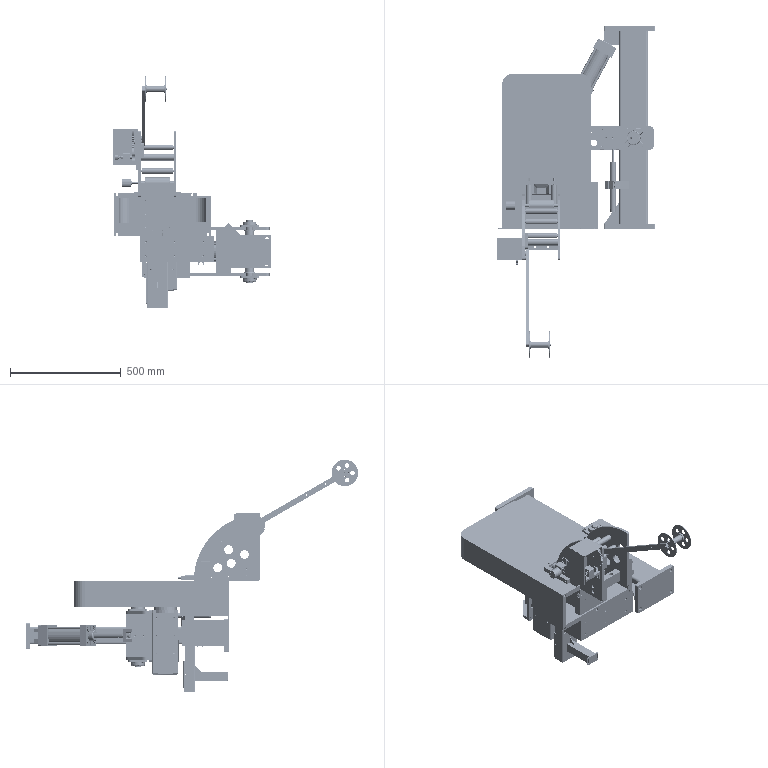Assembly | SolidWorks | mm | 77 component files | 136 solids | 6443 faces | box 714.5 x 1500.09 x 1051.5 mm | volume 27815565 mm3 | plane 2410 | cylinder 2260 | spline 1001 | cone 424 | torus 236 | sphere 112 | commonest cylinder face diameters 5 x141 9 x120 6.8 x118 20 x108 107 x105 102.497 x105 6 x102 4.2 x90
Bill of materials:
320SawBlade | 1 |  | Thin flat circular disc with evenly spaced small teeth or notches around the outer edge and a round hole in the center.
A | 1 |  | Sheet-metal hollow rectangular housing in an L shape (plan view). One end is open with a perimeter flange carrying slotted mounting holes. A long arm runs off to one side and ends in a rounded corner.
B | 1 |  | Sheet-metal shell that wraps a rectangular volume: top panel, two side walls and a partial bottom panel. One end is open, and the bottom has a large curved cutout. A narrow outward lip runs along one lower edge.
CoverPlate | 1 |  | Sheet-metal U-channel: a large flat web with two narrow side flanges bent at roughly 90 degrees. Each flange has one elongated slot.
GuideSlot | 1 |  | Welded or bent sheet bracket. An upright U-channel has a rectangular window near the top. A horizontal arm sticks out from its web, with a triangular gusset underneath and a small end plate carrying two slots.
TransitionPlate | 1 |  | Angle bracket with two legs at about 90 degrees and a rounded bend. The base leg has four round holes in a rectangular pattern, and the upright leg has a chamfered top edge.
AdjustableHydraulicBufferHR60 | 1 |  | Stepped cylindrical pin: a short larger-diameter head at one end, a long main shank, and a much smaller-diameter tip at the other end.
BladeGuard | 1 |  | Plain solid rectangular block (cuboid) with no visible holes or features.
BladeHolder | 1 |  | Flat rectangular bar with two round through-holes near its ends and small corner chamfers on one long edge.
BoltNeedleBearing | 1 |  | Turned stepped part: a large short cylindrical base with a smaller coaxial cylindrical stem. The stem has a narrow circumferential groove partway along it, and the edges are chamfered.
CB-80CylinderFixingBase(DoubleEyelet) | 1 |  | Bracket with a square flange plate, four holes near the corners and a rounded-rectangular central opening. Two parallel lugs stick out from the plate in a clevis-like form, each with an aligned round hole.
ConnectingPin1 | 1 |  | Solid cylindrical pin with chamfered ends and a narrow circumferential groove near each end.
ConnectingPin2 | 1 |  | Solid plain cylinder (pin-like) with a shallow circumferential groove near each end and small edge breaks at both end faces.
CuttingBladeCylinderGasket | 1 |  | L-section angle bracket: a rectangular horizontal plate joined along one long edge to a vertical wall, with a small raised U/C-shaped wall around a rectangular through opening near one corner of the plate.
CuttingBladeModification | 1 |  | Thin flat square plate with two parallel open-ended U-slots entering from one edge and a tapered (wedge-beveled) region along the opposite edge.
CuttingDieMount | 1 |  | Multi-wall block/frame: two parallel side walls bridged by a crossbar on top of a wider base, giving an H-like profile, with a central open cavity, many holes, and a horizontal slot cut partway into one wall.
CuttingDieMountingSeatLocatingBlock | 1 |  | Solid L-shaped block (L outline in plan) with two parallel through holes across one leg.
LocatingStrip | 1 |  | Flat bar of rectangular section with one fully rounded end and a square opposite end, with four through holes in a line along its length.
Mold01-1 | 1 |  | Rectangular block with a tapered (funnel-like) rounded-rectangle through cavity: larger opening on top, smaller opening at bottom, plus a narrow groove across one side face.
'-Mold01-2 | 1 |  | Rectangular block with a straight-walled rounded-rectangle through opening and a narrow groove across one side face; similar to a block with a tapered cavity but with straight walls.
CuttingMotorFixedAxis | 1 |  | Stepped cylindrical shaft: a larger central cylinder with a smaller-diameter coaxial journal extending from each end.
CuttingMotorFixedShaftSleeve | 2 |  | Flanged bushing: a thin wide circular flange on top of a shorter-diameter cylindrical body, with a central through bore.
CylinderMount | 1 |  | Long beam of rectangular section with rectangular end plates at both ends; each end plate has rounded corners and four corner holes; the beam has a central through hole on top, two tiny holes, and a small side tab with a hole near one end.
DamperMountingBlock | 1 |  | Bracket with an inclined arm containing a large bore and a split slot (clamp-style), a horizontal foot with two holes, and a vertical leg with a hole, joined at a filleted corner.
GraphiteCopperSleeve1 | 2 |  | Short plain cylindrical ring or spacer with a concentric through bore; axial length is less than outside diameter.
GraphiteCopperSleeve2- | 1 |  | Plain cylindrical sleeve or spacer with a concentric through bore; axial length is about equal to or slightly more than outside diameter.
ConnectingRod | 1 |  | Solid cylindrical rod or pin with small chamfers at both ends and a small central axial hole in at least one end face.
E6B2-CWZ1XEncoder | 1 |  | Cylindrical housing-like body. One end face has a concentric stepped pilot boss and a small-diameter output shaft; the shaft appears to have a flat or step near its tip. Three small holes are spaced around the end face.
EncoderRoller | 1 |  | Thin-walled cylindrical tube open at both ends with a uniform outer diameter.
EncoderSupport | 1 |  | Bent sheet-like bracket with a Z or joggle profile: two parallel flanges offset by a connecting web. One flange has two parallel obround slots; the other has a large round hole and three small holes around it. The flange ends are rounded.
GuideSeatFixingPlate | 1 |  | Rectangular block with two larger holes through the long face and two smaller holes in one end face.
GuideWheelMountingPlate | 1 |  | Flat plate shaped roughly as a quarter circle with square corners on two sides and one large arc edge. It has many through holes: several large round holes, small round holes, two small obround slots, a narrow slot from the bottom edge, and a rectangular notch at one corner. The rendering shows two identical copies side by side.
LimitPlate1 | 2 |  | Thick rectangular bar with one fully rounded (semicircular) end and one square end, with two in-line obround through slots along its length.
LimitRollerSeat | 2 |  | L-shaped bar of constant thickness with an internal corner fillet. The long leg has a small rectangular side tab or step and a small round through hole near its end; the short leg has an elongated obround through slot.
RollerAxis01 | 1 |  | Long stepped cylindrical shaft with a main central diameter and reduced-diameter shoulders and journals at both ends. One end has two steps down to a small tip; the other end has a single step.
RollerEndCap01 | 1 |  | Flanged hub or bushing: a cylindrical boss with an end chamfer joined to a larger, thin flange, with a central through bore that has a single rectangular keyway.
RollerEndCap02 | 1 |  | Flanged cylindrical bushing: thin circular flange at one end, a shorter-diameter cylindrical body with a small chamfer at the free end, and a central through bore.
'-StainlessSteelRoller(Vertical) | 2 |  | Solid stepped cylindrical shaft/pin: a long large-diameter cylinder, a short intermediate-diameter step, and a smaller-diameter pin extending from one end.
StainlessSteelRoller | 3 |  | Cylindrical roller or pin with rounded/filleted end edges and a short small-diameter stub journal at each end; the stub end face has a small conical center recess.
AdjustmentSeat.1 | 1 |  | L-shaped angle bracket of rectangular cross-section with two parallel elongated slots in the long leg and two parallel slots in the short leg.
AngleDisplacementSensor.1 | 1 |  | Stepped turned shaft/knob: large-diameter cylindrical head with a narrow circumferential groove near one end, followed by a short collar step, an intermediate-diameter section and a smaller-diameter pin with a slot across its end face.
AngleDisplacementSensorMountingPlate.1 | 1 |  | Flat plate with a rectangular lower portion and two chamfered upper corners (pentagon-like outline), one large round hole near the top and two smaller round holes near the bottom corners.
AngleDisplacementSensorNut.1 | 1 |  | Hexagonal ring of uniform thickness with a large plain circular central bore, resembling a thin hex nut shape.
AngleSensorConnectionAxis.1 | 1 |  | Stepped shaft: one end with a radial cross hole and a narrow circumferential groove nearby, a long main section, a larger-diameter collar, and an opposite end section with a flat on its side and a small axial center hole.
BearingHousing.1 | 1 |  | Rectangular block with a large central stepped (counterbored) through hole and four small through holes near the corners.
BearingHousing2.1 | 1 |  | Near-cubic block with two chamfered edges along one side and a central stepped (counterbored) through hole.
CylindricalGear105x1.1 | 1 | 45 | Thin spur gear with many fine teeth around the rim and a central bore with a single keyway notch.
CylindricalGear35x1.1 | 1 | 45 | Wide-face spur gear with roughly thirty-odd straight teeth, a large central bore, and a radial hole passing through the toothed rim.
GuideWheel | 1 |  | Spool-like body: two thin, flat, parallel circular flanges joined by a central cylindrical tube, with a short larger-diameter boss where the tube meets each flange.
GuideWheelAxis | 1 |  | Long, straight, solid cylindrical rod with a narrow ring-shaped groove near each end and a flat machined on one end.
Rolling bearings 6001 GB 276-94 | 4 |  | Ball-bearing-like annular body: concentric outer and inner rings sharing a flat-faced, equal-width profile, with a single row of about 14 spherical balls evenly spaced in the annular gap between them; open faces with no visible shield, seal or cage.
RoundNut.1 | 1 |  | Thick flat ring (annulus) with four rectangular notches evenly spaced around its outer edge.
SwingArm.1 | 1 |  | Long, thin, flat rectangular bar with small through-holes spaced along its length.
SwingRodRotationAxis.1 | 1 |  | Stepped cylindrical shaft with several coaxial diameters and a central bore at the small end.
SwingArmGuard | 1 |  | Thin-walled, sheet-like formed bracket or enclosure: flat top and bottom panels joined by vertical walls, with a perpendicular end flange that has two holes and rounded outer corners.
1 | 1 |  | Rectangular block with an extrusion-like profile: several lengthwise slots and grooves on its outer faces, two large lengthwise through-bores and four smaller corner bores.
2 | 1 |  | Rectangular plate with three parallel cylindrical rods standing out from one face: two long outer rods and a shorter central rod ending in a larger-diameter disc.
3 | 1 |  | Small block body with a lengthwise rounded rib or rod on top between two parallel rails, a stepped lower block, and a cylindrical pin pointing down from one end.
4 | 1 |  | Small block body with a lengthwise cylindrical rod on top between two parallel rails, a lower block section, and a cylindrical pin pointing down from one end.
MotorMount | 1 | Plain Carbon Steel | Plate-built U-shaped frame bracket: a square end plate with two parallel side arms extending from it, an inner cross plate with an angled gusset, and open-ended slots near the free ends of the arms.
SawingMotor | 1 |  | Rectangular housing body with a stepped cylindrical boss on one end, a rectangular box sticking out from one side, and a square flange face with four corner holes.
SC-80X130PistonRod | 1 |  | Long, slender solid cylindrical rod. One end steps down to a short, smaller-diameter cylindrical spigot, with a narrow hexagonal collar (wrench flats) next to it. The far end is plain and appears flat or slightly rounded.
SC-80X130-S-BCylinder | 1 |  | Tie-rod-style cylinder body. A cylindrical barrel sits between two rectangular end blocks, which are held by four slender rods running along the outside. One end block has a protruding round boss with a central through-bore. Its outer face has four small holes at the corners, a shallow recessed outline, and faint diagonal and centre lines.
SC-80X130-S-BCylinderY-Joint | 1 |  | U-shaped clevis block. Two parallel flat prongs with rounded ends are joined by a solid rectangular base. The prongs share one aligned cross-hole. A second hole passes through the base at right angles, opening into the slot between the prongs.
ToolHolder | 1 |  | Flat rectangular plate with small chamfered corners and four through-holes near the corners. A narrow rectangular tab or rib projects from the back face along part of its length, so the side view is T-shaped.
UCF204D1 | 2 |  | Four-bolt square flange housing with a round central boss. The boss holds an insert with an extended inner collar and a central bore. The square flange has rounded corners, four large through-holes at the corners, and diagonal ribs from the boss to the corners. A small nipple projects from the side of the boss.
Mates:
1. coincident | SC-80X130-S-BCylinder-1 face at (-106.845, 345.63, 947) dir (0.479, 0.8778, 0) | CB-80CylinderFixingBase(DoubleEyelet)-1 face at (-148.101, 368.145, 900) dir (-0.479, -0.8778, 0)
2. concentric | SC-80X130-S-BCylinder-1 face at (-184.333, 374.816, 935) dir (0.479, 0.8778, 0) r 5.5 | CB-80CylinderFixingBase(DoubleEyelet)-1 face at (-172.118, 397.2, 935) dir (0.479, 0.8778, 0) r 8.5
3. concentric | SC-80X130-S-BCylinder-1 face at (-184.333, 374.816, 865) dir (0.479, 0.8778, 0) r 5.5 | CB-80CylinderFixingBase(DoubleEyelet)-1 face at (-172.118, 397.2, 865) dir (0.479, 0.8778, 0) r 8.5
4. concentric | CylinderMount-1 face at (-132.772, 396.234, 916) dir (0, 0, -1) r 14 | CB-80CylinderFixingBase(DoubleEyelet)-1 face at (-132.772, 396.234, 865.5) dir (0, 0, 1) r 10
5. concentric | SC-80X130-S-BCylinder-1 face at (-173.49, 321.621, 900) dir (-0.479, -0.8778, 0) r 12.5 | SC-80X130PistonRod-1 face at (-355.042, -11.064, 900) dir (0.479, 0.8778, 0) r 12.5
6. distance | SC-80X130PistonRod-1 face at (-323.95, 33.486, 889.008) dir (-0.479, -0.8778, 0) | SC-80X130-S-BCylinder-1 face at (-269.296, 146.062, 900) dir (-0.479, -0.8778, 0)
7. width | MotorMount-1 face at (67.336, 5.548, 802) dir (0, 0, 1) | MotorMount-1 face at (67.336, 5.548, 998) dir (0, 0, -1) | CylinderMount-1 face at (-77.772, 438.234, 860) dir (0, 0, -1) | CylinderMount-1 face at (-77.772, 438.234, 940) dir (0, 0, 1)
8. width | 320SawBlade-1 face at (-393.08, -172.058, 1071) dir (0, 0, 1) | 320SawBlade-1 face at (-393.08, -172.058, 1068) dir (0, 0, -1) | SawingMotor-1 face at (-418.028, -170.45, 1071) dir (0, 0, -1) | SawingMotor-1 face at (-365.029, -170.559, 1068) dir (0, 0, 1)
9. concentric | SawingMotor-1 face at (-418.028, -170.45, 1100) dir (0, 0, 1) r 42.5 | 320SawBlade-1 face at (-418.028, -170.45, 909.976) dir (0, 0, -1) r 25
10. concentric | SC-80X130PistonRod-1 face at (-339.234, 17.903, 900) dir (-0.479, -0.8778, 0) r 10 | SC-80X130-S-BCylinderY-Joint-1 face at (-344.024, 9.125, 900) dir (0.479, 0.8778, 0) r 10.05
11. coincident | SC-80X130PistonRod-1 face at (-344.024, 9.125, 900) dir (-0.479, -0.8778, 0) | SC-80X130-S-BCylinderY-Joint-1 face at (-324.274, -1.653, 930) dir (0.479, 0.8778, 0)
12. width | SC-80X130-S-BCylinderY-Joint-1 face at (-364.991, -76.266, 930) dir (0, 0, 1) | SC-80X130-S-BCylinderY-Joint-1 face at (-324.274, -1.653, 870) dir (0, 0, -1) | MotorMount-1 face at (-220.272, -46.358, 885) dir (0, 0, -1) | MotorMount-1 face at (-220.272, -46.358, 915) dir (0, 0, 1)
13. concentric | MotorMount-1 face at (-372.766, -43.543, 750) dir (0, 0, 1) r 14 | SC-80X130-S-BCylinderY-Joint-1 face at (-372.766, -43.543, 930) dir (0, 0, -1) r 14
14. coincident | MotorMount-1 face at (67.336, 5.548, 1010) dir (0, 0, 1) | UCF204D1-1 face at (-54.706, -14.7, 1010) dir (0, 0, -1)
15. concentric | MotorMount-1 face at (-22.772, -46.766, 750) dir (0, 0, 1) r 15 | UCF204D1-1 face at (-22.772, -46.766, 1010) dir (0, 0, -1) r 10
16. concentric | CylinderMount-1 face at (-22.772, -46.766, 824) dir (0, 0, 1) r 19 | MotorMount-1 face at (-22.772, -46.766, 750) dir (0, 0, 1) r 15
17. concentric | MotorMount-1 face at (-54.706, -14.7, 1010) dir (0, 0, 1) r 4.25 | UCF204D1-1 face at (-54.706, -14.7, 1019.35) dir (0, 0, -1) r 6
18. coincident | MotorMount-1 face at (67.336, 5.548, 790) dir (0, 0, -1) | UCF204D1-2 face at (9.294, -14.832, 790) dir (0, 0, 1)
19. concentric | MotorMount-1 face at (9.294, -14.832, 1010) dir (0, 0, 1) r 4.25 | UCF204D1-2 face at (9.294, -14.832, 780.65) dir (0, 0, 1) r 6
20. concentric | MotorMount-1 face at (-54.706, -14.7, 1010) dir (0, 0, 1) r 4.25 | UCF204D1-2 face at (-54.706, -14.7, 780.65) dir (0, 0, 1) r 6
21. concentric | CylinderMount-1 face at (-22.772, -46.766, 824) dir (0, 0, 1) r 19 | CuttingMotorFixedAxis-1 face at (-22.772, -46.766, 442.271) dir (0, 0, -1) r 19
22. width | CuttingMotorFixedAxis-1 face at (-22.772, -36.766, 806) dir (0, 0, -1) | CuttingMotorFixedAxis-1 face at (-22.772, -27.766, 994) dir (0, 0, 1) | CylinderMount-1 face at (-77.772, 438.234, 940) dir (0, 0, 1) | CylinderMount-1 face at (-77.772, 438.234, 860) dir (0, 0, -1)
23. coincident | CuttingMotorFixedAxis-1 face at (-22.772, -36.766, 806) dir (0, 0, -1) | CuttingMotorFixedShaftSleeve-1 face at (-12.772, -46.766, 806) dir (0, 0, 1)
24. concentric | CuttingMotorFixedAxis-1 face at (-22.772, -46.766, 442.271) dir (0, 0, -1) r 10 | CuttingMotorFixedShaftSleeve-1 face at (-22.772, -46.766, -457.669) dir (0, 0, -1) r 15
25. coincident | CuttingMotorFixedAxis-1 face at (-22.772, -27.766, 994) dir (0, 0, 1) | CuttingMotorFixedShaftSleeve-2 face at (-32.009, -50.596, 994) dir (0, 0, -1)
26. concentric | CuttingMotorFixedAxis-1 face at (-22.772, -46.766, 442.271) dir (0, 0, -1) r 10 | CuttingMotorFixedShaftSleeve-2 face at (-22.772, -46.766, 2257.669) dir (0, 0, 1) r 15
27. width | ConnectingPin1-1 face at (-372.766, -43.543, 933) dir (0, 0, 1) | ConnectingPin1-1 face at (-372.766, -43.543, 867) dir (0, 0, -1) | SC-80X130-S-BCylinderY-Joint-1 face at (-324.274, -1.653, 870) dir (0, 0, -1) | SC-80X130-S-BCylinderY-Joint-1 face at (-364.991, -76.266, 930) dir (0, 0, 1)
28. concentric | SC-80X130-S-BCylinderY-Joint-1 face at (-372.766, -43.543, 930) dir (0, 0, -1) r 14 | ConnectingPin1-1 face at (-372.766, -43.543, 933) dir (0, 0, -1) r 10
29. concentric | SC-80X130-S-BCylinderY-Joint-1 face at (-372.766, -43.543, 930) dir (0, 0, -1) r 14 | GraphiteCopperSleeve1-1 face at (-372.766, -43.543, 930) dir (0, 0, -1) r 14
30. coincident | SC-80X130-S-BCylinderY-Joint-1 face at (-331.459, -14.82, 915) dir (0, 0, -1) | GraphiteCopperSleeve1-1 face at (-372.766, -43.543, 915) dir (0, 0, -1)
31. concentric | SC-80X130-S-BCylinderY-Joint-1 face at (-372.766, -43.543, 930) dir (0, 0, -1) r 14 | GraphiteCopperSleeve1-2 face at (-372.766, -43.543, 885) dir (0, 0, -1) r 14
32. coincident | SC-80X130-S-BCylinderY-Joint-1 face at (-364.991, -76.266, 885) dir (0, 0, 1) | GraphiteCopperSleeve1-2 face at (-372.766, -43.543, 885) dir (0, 0, 1)
33. coincident | MotorMount-1 face at (-220.272, -46.358, 885) dir (0, 0, -1) | GraphiteCopperSleeve2--1 face at (-372.766, -43.543, 885) dir (0, 0, -1)
34. concentric | MotorMount-1 face at (-372.766, -43.543, 750) dir (0, 0, 1) r 14 | GraphiteCopperSleeve2--1 face at (-372.766, -43.543, 915) dir (0, 0, -1) r 14
35. coincident | MotorMount-1 face at (67.336, 5.548, 998) dir (0, 0, -1) | BoltNeedleBearing-1 face at (-115.847, -83.074, 998) dir (0, 0, 1)
36. concentric | MotorMount-1 sketch segment at (-115.847, -83.074, 1010) dir (0, 0, 1) r 5.5 | BoltNeedleBearing-1 face at (-115.847, -83.074, 1021) dir (0, 0, -1) r 5
37. distance | CylinderMount-1 face at (-41.272, -436.766, 900) dir (0, 1, 0) | AdjustableHydraulicBufferHR60-1 face at (-115.446, -379.666, 991.405) dir (0, -1, 0)
38. concentric | CylinderMount-1 face at (-25.272, -249.266, 940) dir (0, 0, 1) r 2.5 | DamperMountingBlock-2 face at (-25.272, -249.266, 955) dir (0, 0, 1) r 3.5
39. coincident | CylinderMount-1 face at (-77.772, 438.234, 940) dir (0, 0, 1) | DamperMountingBlock-2 face at (-7.272, -241.766, 940) dir (0, 0, -1)
40. concentric | CylinderMount-1 face at (-25.272, -269.266, 940) dir (0, 0, 1) r 2.5 | DamperMountingBlock-2 face at (-25.272, -269.266, 955) dir (0, 0, 1) r 5.5
41. concentric | AdjustableHydraulicBufferHR60-1 face at (-115.446, -156.166, 991.405) dir (0, -1, 0) r 12 | DamperMountingBlock-2 face at (-115.446, -241.766, 991.405) dir (0, -1, 0) r 12
42. concentric | CB-80CylinderFixingBase(DoubleEyelet)-1 face at (-132.772, 396.234, 865.5) dir (0, 0, 1) r 10 | ConnectingPin2-1 face at (-132.772, 396.234, 937.5) dir (0, 0, -1) r 10
43. width | ConnectingPin2-1 face at (-132.772, 396.234, 937.5) dir (0, 0, 1) | ConnectingPin2-1 face at (-132.772, 396.234, 862.5) dir (0, 0, -1) | CB-80CylinderFixingBase(DoubleEyelet)-1 face at (-143.049, 425.766, 868) dir (0, 0, -1) | CB-80CylinderFixingBase(DoubleEyelet)-1 face at (-143.049, 425.766, 932) dir (0, 0, 1)
44. coincident | MotorMount-1 face at (-220.405, -110.858, 900) dir (-0.002066, -1, 0) | SawingMotor-1 face at (-352.905, -110.584, 723) dir (0.002066, 1, 0)
45. distance | SawingMotor-1 face at (-485.911, -113.309, 723) dir (-1, 0.002066, 0) | MotorMount-1 face at (-507.904, -110.264, 780) dir (-1, 0.002066, 0)
46. distance | SawingMotor-1 face at (-377.915, -115.532, 1015) dir (0, 0, 1) | MotorMount-1 face at (-327.905, -110.636, 1017) dir (0, 0, 1)
47. coincident | AA-1/A-1 face at (-636.772, -452.766, 968.5) dir (0, 0, -1) | CuttingBladeCylinderGasket-1 face at (-361.772, -326.766, 968.5) dir (0, 0, 1)
48. width | CuttingBladeModification-1 face at (-464.272, -249.266, 895.2) dir (0, 1, 0) | CuttingBladeModification-1 face at (-464.272, -314.266, 895.2) dir (0, -1, 0) | CuttingDie-1/-Mold01-2-1 face at (-461.272, -261.766, 1002) dir (0, -1, 0) | CuttingDie-1/-Mold01-2-1 face at (-461.272, -301.766, 1002) dir (0, 1, 0)
49. width | BladeGuard-1 face at (-464.272, -246.766, 910.2) dir (0, 1, 0) | BladeGuard-1 face at (-464.272, -316.766, 910.2) dir (0, -1, 0) | CuttingDie-1/-Mold01-2-1 face at (-461.272, -261.766, 1002) dir (0, -1, 0) | CuttingDie-1/-Mold01-2-1 face at (-461.272, -301.766, 1002) dir (0, 1, 0)
50. parallel | CuttingDie-1/-Mold01-2-1 face at (-464.272, -298.766, 1002) dir (1, 0, 0) | BladeGuard-1 face at (-464.272, -316.766, 910.2) dir (1, 0, 0)
51. coincident | CuttingDie-1/-Mold01-2-1 face at (-464.272, -298.766, 1002) dir (1, 0, 0) | BladeGuard-1 face at (-464.272, -316.766, 910.2) dir (1, 0, 0)
52. coincident | CuttingBladeCylinderGasket-1 face at (-479.272, -246.766, 968.5) dir (1, 0, 0) | BladeGuard-1 face at (-479.272, -316.766, 910.2) dir (-1, 0, 0)
53. width | BladeGuard-1 face at (-471.772, -281.766, 910.2) dir (0, 0, 1) | BladeGuard-1 face at (-471.772, -281.766, 880.2) dir (0, 0, -1) | CuttingBladeModification-1 face at (-404.772, -249.266, 894.2) dir (0, 0, -1) | CuttingBladeModification-1 face at (-404.772, -249.266, 896.2) dir (0, 0, 1)
54. parallel | ToolHolder-1 face at (-404.772, -327.766, 894.5) dir (-1, 0, 0) | CuttingBladeModification-1 face at (-404.772, -249.266, 894.2) dir (1, 0, 0)
55. coincident | ToolHolder-1 face at (-404.772, -327.766, 894.5) dir (-1, 0, 0) | CuttingBladeModification-1 face at (-404.772, -249.266, 894.2) dir (1, 0, 0)
56. coincident | ToolHolder-1 face at (-392.772, -327.766, 894.5) dir (1, 0, 0) | MGPM63-55-M9NV_0_1_0-1/2-1 face at (-392.772, -327.766, 894.5) dir (-1, 0, 0)
57. concentric | MGPM63-55-M9NV_0_1_0-1/2-1 face at (-384.772, -392.766, 869.5) dir (1, 0, 0) r 4.188 | ToolHolder-1 face at (-404.772, -392.766, 869.5) dir (-1, 0, 0) r 5.5
58. coincident | AA-1/A-1 face at (-484.272, -253.766, 1166.5) dir (0, -1, 0) | GuideMechanism-1/LimitRollerSeat-2 face at (-413.272, -253.766, 1171.5) dir (0, -1, 0)
59. coincident | AA-1/A-1 face at (-616.772, 243.234, 1146.5) dir (0, 0, 1) | GuideMechanism-1/GuideWheelMountingPlate-1 face at (-353.272, -298.766, 1146.5) dir (0, 0, -1)
60. coincident | A-1 face at (322.308, 345.256, 549.124) dir (0, 0, 1) | TransitionPlate-1 face at (100.308, -237.257, 549.124) dir (0, 0, -1)
61. coincident | A-1 face at (189.808, -201.744, 525.124) dir (0, 1, 0) | TransitionPlate-1 face at (100.308, -201.744, 549.124) dir (0, -1, 0)
62. width | TransitionPlate-1 face at (189.308, -202.744, 548.124) dir (1, 0, 0) | TransitionPlate-1 face at (100.308, -202.744, 552.124) dir (-1, 0, 0) | A-1 face at (189.808, -151.744, 525.124) dir (-1, 0, 0) | A-1 face at (99.808, -151.744, 525.124) dir (1, 0, 0)
63. width | GuideSlot-1 face at (192.808, -151.744, 838.124) dir (1, 0, 0) | GuideSlot-1 face at (96.808, -151.744, 838.124) dir (-1, 0, 0) | A-1 face at (99.808, -151.744, 525.124) dir (1, 0, 0) | A-1 face at (189.808, -151.744, 525.124) dir (-1, 0, 0)
64. coincident | GuideSlot-1 face at (189.808, -151.744, 838.124) dir (0, 1, 0) | CoverPlate-1 face at (144.808, -151.744, 968.124) dir (0, -1, 0)
65. width | CoverPlate-1 face at (96.808, -150.244, 968.124) dir (1, 0, 0) | CoverPlate-1 face at (192.808, -150.244, 968.124) dir (-1, 0, 0) | GuideSlot-1 face at (96.808, -151.744, 838.124) dir (-1, 0, 0) | GuideSlot-1 face at (192.808, -151.744, 838.124) dir (1, 0, 0)
66. distance | A-1 face at (322.308, 345.256, 703.124) dir (0, 0, 1) | CoverPlate-1 face at (97.808, -151.744, 908.124) dir (0, 0, -1)
67. coincident | A-1 face at (122.308, 345.256, 624.124) dir (0, 1, 0) | B-1 face at (322.308, 345.256, 663.124) dir (0, 1, 0)
68. coincident | A-1 face at (92.308, -107.744, 699.124) dir (1, 0, 0) | B-1 face at (92.308, 103.756, 604.124) dir (-1, 0, 0)
69. coincident | A-1 face at (322.308, 345.256, 545.124) dir (0, 0, -1) | B-1 face at (322.308, -137.744, 545.124) dir (0, 0, -1)
70. parallel | A-1 face at (322.308, 345.256, 545.124) dir (0, 0, -1) | AA plane at (0, 0, 0) dir (0, 0, 1)
71. parallel | A-1 face at (122.308, -354.744, 624.124) dir (0, -1, 0) | AA plane at (0, 0, 0) dir (0, 1, 0)
72. distance | GuideSlot-1 face at (100.808, -200.744, 838.124) dir (0, 0, -1) | A-1 face at (322.308, 345.256, 703.124) dir (0, 0, 1)
73. coincident | CuttingDieMount-1 face at (49.289, -80.571, 190) dir (1, 0, 0) | CuttingDieMountingSeatLocatingBlock-1 face at (49.289, -50.571, 120.5) dir (1, 0, 0)
74. coincident | CuttingDieMount-1 face at (49.289, -95.571, 102.5) dir (0, 0, -1) | CuttingDieMountingSeatLocatingBlock-1 face at (49.289, -95.571, 102.5) dir (0, 0, 1)
75. coincident | CuttingDieMount-1 face at (49.289, -65.571, 102.5) dir (0, 1, 0) | CuttingDieMountingSeatLocatingBlock-1 face at (49.289, -65.571, 102.5) dir (0, -1, 0)
76. coincident | CuttingDieMount-1 face at (29.289, -95.571, 102.5) dir (-1, 0, 0) | LocatingStrip-1 face at (29.289, -95.571, 282.5) dir (1, 0, 0)
77. coincident | CuttingDieMount-1 face at (4.289, -83.571, 102.5) dir (0, -1, 0) | LocatingStrip-1 face at (29.289, -83.571, 282.5) dir (0, 1, 0)
78. coincident | CuttingDieMount-1 face at (49.289, -95.571, 102.5) dir (0, 0, -1) | LocatingStrip-1 face at (16.789, -89.571, 102.5) dir (0, 0, -1)
79. coincident | CuttingDieMount-1 face at (-20.711, 54.429, 190) dir (0, 1, 0) | -Mold01-2-1 face at (-55.711, 54.429, 190) dir (0, -1, 0)
80. width | -Mold01-2-1 face at (-53.211, 54.429, 142) dir (-1, 0, 0) | -Mold01-2-1 face at (-58.211, 54.429, 142) dir (1, 0, 0) | CuttingDieMount-1 face at (-58.211, 24.429, 139.5) dir (-1, 0, 0) | CuttingDieMount-1 face at (-53.211, 24.429, 139.5) dir (1, 0, 0)
81. coincident | CuttingDieMount-1 face at (-90.711, 99.429, 142) dir (0, 0, 1) | -Mold01-2-1 face at (-88.211, 119.429, 142) dir (0, 0, -1)
82. coincident | CuttingDieMount-1 face at (-20.711, 54.429, 190) dir (0, 1, 0) | Mold01-1-3 face at (14.289, 54.429, 190) dir (0, -1, 0)
83. width | Mold01-1-3 face at (11.789, 54.429, 142) dir (1, 0, 0) | Mold01-1-3 face at (16.789, 54.429, 142) dir (-1, 0, 0) | CuttingDieMount-1 face at (11.789, 24.429, 139.5) dir (-1, 0, 0) | CuttingDieMount-1 face at (16.789, 24.429, 139.5) dir (1, 0, 0)
84. coincident | CuttingDieMount-1 face at (-90.711, 99.429, 142) dir (0, 0, 1) | Mold01-1-3 face at (-18.211, 119.429, 142) dir (0, 0, -1)
85. width | GuideSeatFixingPlate-1 face at (16.59, -118.843, 215) dir (1, 0, 0) | GuideSeatFixingPlate-1 face at (-131.41, -118.843, 215) dir (-1, 0, 0) | GuideWheelMountingPlate-1 face at (16.59, -163.843, 150) dir (-1, 0, 0) | GuideWheelMountingPlate-1 face at (-131.41, -163.843, 150) dir (1, 0, 0)
86. distance | GuideWheelMountingPlate-1 face at (28.59, 136.157, 150) dir (0, 0, -1) | GuideSeatFixingPlate-1 face at (-57.41, -103.843, 165) dir (0, 0, -1)
87. distance | GuideWheelMountingPlate-1 face at (28.59, -163.843, 150) dir (0, -1, 0) | GuideSeatFixingPlate-1 face at (16.59, -118.843, 215) dir (0, -1, 0)
88. concentric | GuideWheelMountingPlate-1 face at (20.59, -83.843, 330) dir (1, 0, 0) r 7 | ConnectingRod-1 face at (16.59, -83.843, 330) dir (-1, 0, 0) r 15
89. coincident | GuideWheelMountingPlate-1 face at (16.59, -163.843, 150) dir (-1, 0, 0) | ConnectingRod-1 face at (16.59, -83.843, 330) dir (1, 0, 0)
90. width | LimitRollerSeat-1 face at (-123.41, 128.657, 175) dir (0, 0, 1) | LimitRollerSeat-1 face at (-123.41, 128.657, 155) dir (0, 0, -1) | GuideWheelMountingPlate-1 face at (28.59, 154.061, 155) dir (0, 0, 1) | GuideWheelMountingPlate-1 face at (28.59, 154.061, 175) dir (0, 0, -1)
91. coincident | GuideWheelMountingPlate-1 face at (-143.41, -163.843, 150) dir (-1, 0, 0) | LimitRollerSeat-1 face at (-143.41, 86.157, 155) dir (1, 0, 0)
92. coincident | GuideWheelMountingPlate-1 face at (28.59, -163.843, 150) dir (1, 0, 0) | LimitRollerSeat-2 face at (28.59, 86.157, 175) dir (-1, 0, 0)
93. coincident | GuideWheelMountingPlate-1 face at (28.59, 154.061, 155) dir (0, 0, 1) | LimitRollerSeat-2 face at (8.59, 128.657, 155) dir (0, 0, -1)
94. coincident | GuideWheelMountingPlate-1 face at (28.59, 66.157, 155) dir (0, 1, 0) | LimitRollerSeat-1 face at (-163.41, 66.157, 175) dir (0, -1, 0)
95. coincident | GuideWheelMountingPlate-1 face at (28.59, 66.157, 155) dir (0, 1, 0) | LimitRollerSeat-2 face at (48.59, 66.157, 155) dir (0, -1, 0)
96. width | -StainlessSteelRoller(Vertical)-7 face at (-130.184, 181.157, 169) dir (0, 0, 1) | -StainlessSteelRoller(Vertical)-7 face at (-125.226, 181.157, 161) dir (0, 0, -1) | LimitRollerSeat-1 face at (-93.41, 41.157, 161) dir (0, 0, 1) | LimitRollerSeat-1 face at (-93.41, 41.157, 169) dir (0, 0, -1)
97. coincident | LimitRollerSeat-1 face at (-83.41, 181.157, 155) dir (0, -1, 0) | -StainlessSteelRoller(Vertical)-7 face at (-114.91, 181.157, 165) dir (0, 1, 0)
98. coincident | LimitRollerSeat-2 face at (-21.41, 41.157, 161) dir (0, 0, 1) | -StainlessSteelRoller(Vertical)-8 face at (15.363, 181.157, 161) dir (0, 0, -1)
99. coincident | LimitRollerSeat-2 face at (-31.41, 181.157, 175) dir (0, -1, 0) | -StainlessSteelRoller(Vertical)-8 face at (0.08965, 181.157, 165) dir (0, 1, 0)
100. distance | -StainlessSteelRoller(Vertical)-7 plane at (-114.91, 125.157, 165) dir (-1, 0, 0) | -StainlessSteelRoller(Vertical)-8 plane at (0.08965, 125.157, 165) dir (1, 0, 0)
101. width | -StainlessSteelRoller(Vertical)-7 plane at (-114.91, 125.157, 165) dir (-1, 0, 0) | -StainlessSteelRoller(Vertical)-8 plane at (0.08965, 125.157, 165) dir (1, 0, 0) | LimitRollerSeat-2 face at (48.59, 191.157, 155) dir (1, 0, 0) | LimitRollerSeat-1 face at (-163.41, 191.157, 175) dir (-1, 0, 0)
102. concentric | GuideWheelMountingPlate-1 face at (-131.41, 56.894, 267.368) dir (-1, 0, 0) r 3 | StainlessSteelRoller-3 face at (-277.595, 56.894, 267.368) dir (-1, 0, 0) r 12.5
103. concentric | GuideWheelMountingPlate-1 face at (-131.41, 9.821, 329.835) dir (-1, 0, 0) r 3 | StainlessSteelRoller-4 face at (-277.595, 9.821, 329.835) dir (-1, 0, 0) r 12.5
104. concentric | GuideWheelMountingPlate-1 face at (-131.41, -54.25, 374.699) dir (-1, 0, 0) r 3 | StainlessSteelRoller-2 face at (-277.595, -54.25, 374.699) dir (-1, 0, 0) r 12.5
105. coincident | GuideWheelMountingPlate-1 face at (-131.41, -163.843, 150) dir (1, 0, 0) | StainlessSteelRoller-4 face at (-131.41, 9.821, 329.835) dir (-1, 0, 0)
106. coincident | StainlessSteelRoller-2 face at (12.59, -41.758, 374.249) dir (1, 0, 0) | StainlessSteelRoller-4 face at (12.59, 21.948, 326.801) dir (1, 0, 0)
107. coincident | GuideWheelMountingPlate-1 face at (-143.41, -163.843, 150) dir (-1, 0, 0) | SwingArm-1/AdjustmentSeat.1-1 face at (-143.41, -116.343, 269.95) dir (1, 0, 0)
108. distance | GuideWheelMountingPlate-1 face at (-131.41, 136.157, 150) dir (0, 0, -1) | SwingArm-1/AdjustmentSeat.1-1 face at (-153.41, -116.343, 269.95) dir (0, 0, -1)
109. concentric | GuideWheelMountingPlate-1 face at (-143.41, 82.359, 213.412) dir (1, 0, 0) r 7.5 | EncoderRoller-1 face at (-428.401, 82.359, 213.412) dir (-1, 0, 0) r 26
110. concentric | EncoderRoller-1 face at (-428.401, 82.359, 213.412) dir (-1, 0, 0) r 26 | RollerAxis01-1 face at (466.097, 82.359, 213.412) dir (1, 0, 0) r 7.5
111. concentric | EncoderRoller-1 edge at (-109.91, 82.359, 213.412) dir (-1, 0, 0) r 26 | RollerEndCap02-1 face at (-114.91, 82.359, 213.412) dir (-1, 0, 0) r 22.5
112. coincident | EncoderRoller-1 face at (-109.91, 77.902, 209.395) dir (-1, 0, 0) | RollerEndCap02-1 face at (-109.91, 59.859, 213.412) dir (1, 0, 0)
113. concentric | EncoderRoller-1 face at (-19.91, 82.359, 213.412) dir (1, 0, 0) r 22.5 | RollerEndCap01-1 face at (0.08965, 82.359, 213.412) dir (1, 0, 0) r 22.5
114. coincident | EncoderRoller-1 face at (-4.91, 63.047, 196.003) dir (1, 0, 0) | RollerEndCap01-1 face at (-4.91, 104.859, 213.412) dir (-1, 0, 0)
115. coincident | RollerAxis01-1 face at (-114.91, 82.359, 213.412) dir (-1, 0, 0) | RollerEndCap02-1 face at (-114.91, 56.359, 213.412) dir (-1, 0, 0)
116. width | RollerEndCap01-1 face at (0.08965, 108.359, 213.412) dir (1, 0, 0) | RollerEndCap02-1 face at (-114.91, 56.359, 213.412) dir (-1, 0, 0) | GuideWheelMountingPlate-1 face at (-143.41, -163.843, 150) dir (-1, 0, 0) | GuideWheelMountingPlate-1 face at (28.59, -163.843, 150) dir (1, 0, 0)
117. concentric | RollerAxis01-1 face at (-141.41, 82.359, 213.412) dir (-1, 0, 0) r 3 | E6B2-CWZ1XEncoder-1 face at (-158.41, 82.359, 213.412) dir (-1, 0, 0) r 3
118. parallel | GuideWheelMountingPlate-1 face at (-131.41, -163.843, 150) dir (0, -1, 0) | E6B2-CWZ1XEncoder-1 face at (-168.41, 84.359, 215.648) dir (0, 1, 0)
119. coincident | E6B2-CWZ1XEncoder-1 face at (-178.41, 82.359, 213.412) dir (1, 0, 0) | EncoderSupport-1 face at (-178.41, 102.359, 193.412) dir (-1, 0, 0)
120. concentric | E6B2-CWZ1XEncoder-1 face at (-178.41, 82.359, 213.412) dir (-1, 0, 0) r 20 | EncoderSupport-1 face at (-168.41, 82.359, 213.412) dir (-1, 0, 0) r 10.1
121. parallel | GuideWheelMountingPlate-1 face at (-131.41, -163.843, 150) dir (0, -1, 0) | EncoderSupport-1 face at (-178.41, 102.359, 237.675) dir (0, 1, 0)
122. distance | RollerAxis01-1 face at (-156.41, 89.324, 216.194) dir (-1, 0, 0) | E6B2-CWZ1XEncoder-1 face at (-158.41, 82.359, 213.412) dir (1, 0, 0)
123. distance | GuideWheelMountingPlate-1 face at (-131.41, -163.843, 150) dir (0, -1, 0) | SwingArm-1/BearingHousing.1-1 face at (-143.41, -153.843, 430) dir (0, -1, 0)
124. coincident | GuideWheelMountingPlate-1 face at (-131.41, -163.843, 150) dir (1, 0, 0) | LimitPlate1-1 face at (-131.41, -153.843, 360.5) dir (-1, 0, 0)
125. coincident | GuideWheelMountingPlate-1 face at (-131.41, -163.843, 150) dir (0, -1, 0) | LimitPlate1-1 face at (-116.41, -163.843, 395.5) dir (0, -1, 0)
126. distance | LimitPlate1-1 face at (-116.41, -163.843, 325.5) dir (0, 0, -1) | GuideWheelMountingPlate-1 face at (-131.41, 136.157, 150) dir (0, 0, -1)
127. coincident | GuideWheelMountingPlate-1 face at (-131.41, -163.843, 150) dir (1, 0, 0) | LimitPlate1-2 face at (-131.41, -78.843, 415) dir (-1, 0, 0)
128. distance | GuideWheelMountingPlate-1 face at (-131.41, -163.843, 150) dir (0, -1, 0) | LimitPlate1-2 face at (-116.41, -43.843, 405) dir (0, 1, 0)
129. distance | LimitPlate1-2 face at (-116.41, -113.843, 405) dir (0, 0, -1) | GuideWheelMountingPlate-1 face at (-131.41, 136.157, 150) dir (0, 0, -1)
130. angle | GuideWheelMountingPlate-1 face at (-131.41, -163.843, 150) dir (0, -1, 0) | SwingArm-1/SwingArm.1-1 face at (-124.91, -560.115, 631.675) dir (0, -0.5, -0.866)
131. coincident | GuideWheelMountingPlate-1 face at (-143.41, -163.843, 150) dir (-1, 0, 0) | SwingArmGuard-1 face at (-143.41, -55.343, 376.5) dir (1, 0, 0)
132. distance | SwingArmGuard-1 face at (-144.91, -55.343, 455) dir (0, 0, -1) | GuideWheelMountingPlate-1 face at (-131.41, -163.843, 150) dir (-1, 0, 0) r 300
133. coincident | GuideWheelMountingPlate-1 face at (-131.41, -163.843, 150) dir (0, -1, 0) | SwingArmGuard-1 face at (-145.647, -163.843, 456.5) dir (0, -1, 0)
134. concentric | BearingHousing2.1-1 face at (-11.692, 4.23, 47) dir (0, 0, 1) r 14 | Rolling bearings 6001 GB 276-94-1 face at (-11.692, 4.23, 44.029) dir (0, 0, -1) r 6
135. coincident | BearingHousing2.1-1 face at (-11.692, 4.23, 47) dir (0, 0, 1) | Rolling bearings 6001 GB 276-94-1 face at (-11.692, 18.23, 47) dir (0, 0, -1)
136. concentric | BearingHousing2.1-1 face at (-11.692, 4.23, 33) dir (0, 0, -1) r 14 | Rolling bearings 6001 GB 276-94-2 face at (-11.692, 4.23, 20.289) dir (0, 0, -1) r 14
137. coincident | BearingHousing2.1-1 face at (-11.692, 4.23, 33) dir (0, 0, -1) | Rolling bearings 6001 GB 276-94-2 face at (-11.692, 18.23, 33) dir (0, 0, 1)
138. concentric | Rolling bearings 6001 GB 276-94-1 face at (-11.692, 4.23, 44.029) dir (0, 0, -1) r 6 | AngleSensorConnectionAxis.1-1 face at (-11.692, 4.23, 65) dir (0, 0, -1) r 6
139. coincident | Rolling bearings 6001 GB 276-94-2 face at (-11.692, 12.897, 25) dir (0, 0, -1) | AngleSensorConnectionAxis.1-1 face at (-11.692, 4.23, 25) dir (0, 0, 1)
140. parallel | BearingHousing2.1-1 face at (-31.692, 21.73, 55) dir (0, 1, 0) | AngleSensorConnectionAxis.1-1 face at (-8.376, 9.23, 19.708) dir (0, 1, 0)
141. concentric | AngleSensorConnectionAxis.1-1 face at (-11.692, 4.23, 65) dir (0, 0, -1) r 6 | AngleDisplacementSensor.1-1 face at (-11.692, 4.23, 58) dir (0, 0, 1) r 3
142. concentric | AngleDisplacementSensor.1-1 face at (-11.692, 4.23, 58) dir (0, 0, 1) r 3 | AngleDisplacementSensorMountingPlate.1-1 face at (-11.692, 4.23, 75) dir (0, 0, 1) r 6
143. coincident | AngleDisplacementSensor.1-1 face at (-11.692, 4.23, 78) dir (0, 0, -1) | AngleDisplacementSensorMountingPlate.1-1 face at (-1.692, 4.23, 78) dir (0, 0, 1)
144. concentric | AngleDisplacementSensor.1-1 face at (-11.692, 4.23, 70) dir (0, 0, 1) r 5 | AngleDisplacementSensorNut.1-1 face at (-11.692, 4.23, 72) dir (0, 0, -1) r 5.05
145. coincident | AngleDisplacementSensorMountingPlate.1-1 face at (-1.692, 4.23, 75) dir (0, 0, -1) | AngleDisplacementSensorNut.1-1 face at (-11.692, 4.23, 75) dir (0, 0, 1)
146. coincident | AngleDisplacementSensorMountingPlate.1-1 face at (-1.692, 4.23, 75) dir (0, 0, -1) | AdjustmentSeat.1-1 face at (8.308, -13.27, 75) dir (0, 0, 1)
147. concentric | AngleDisplacementSensorMountingPlate.1-1 face at (13.308, -5.77, 75) dir (0, 0, 1) r 2.75 | AdjustmentSeat.1-1 face at (13.308, -5.77, 75) dir (0, 0, 1) r 2.1
148. concentric | AngleDisplacementSensorMountingPlate.1-1 face at (13.308, 14.23, 75) dir (0, 0, 1) r 2.75 | AdjustmentSeat.1-1 face at (13.308, 14.23, 75) dir (0, 0, 1) r 2.1
149. coincident | BearingHousing2.1-1 face at (8.308, 21.73, 55) dir (1, 0, 0) | AdjustmentSeat.1-1 face at (8.308, -13.27, -15) dir (-1, 0, 0)
150. distance | BearingHousing2.1-1 face at (-11.692, 4.23, 55) dir (0, 0, 1) | AngleDisplacementSensorMountingPlate.1-1 face at (-1.692, 4.23, 75) dir (0, 0, -1)
151. concentric | AngleSensorConnectionAxis.1-1 face at (-11.692, 4.23, 13) dir (0, 0, -1) r 6 | CylindricalGear35x1.1-1 face at (-11.692, 4.23, -2) dir (0, 0, 1) r 6
152. coincident | AngleSensorConnectionAxis.1-1 face at (-11.692, 4.23, 13) dir (0, 0, -1) | CylindricalGear35x1.1-1 face at (-11.692, 4.23, 13) dir (0, 0, 1)
153. coincident | CylindricalGear35x1.1-1 face at (-11.692, 4.23, 13) dir (0, 0, 1) | CylindricalGear105x1.1-1 face at (-81.742, 4.23, 13) dir (0, 0, 1)
154. coincident | CylindricalGear35x1.1-1 plane at (-11.692, 4.23, -2) dir (0, 1, 0) | CylindricalGear105x1.1-1 plane at (-81.742, 4.23, 3) dir (0, 1, 0)
155. distance | CylindricalGear35x1.1-1 plane at (-11.692, 4.23, -2) dir (1, 0, 0) | CylindricalGear105x1.1-1 plane at (-81.742, 4.23, 3) dir (1, 0, 0)
156. concentric | CylindricalGear105x1.1-1 face at (-81.742, 4.23, 13) dir (0, 0, -1) r 8 | SwingRodRotationAxis.1-1 face at (-81.742, 4.23, 13) dir (0, 0, -1) r 8
157. coincident | CylindricalGear105x1.1-1 face at (-81.742, 4.23, 3) dir (0, 0, -1) | SwingRodRotationAxis.1-1 face at (-81.742, 4.23, 3) dir (0, 0, 1)
158. parallel | BearingHousing2.1-1 face at (-31.692, 21.73, 55) dir (0, 1, 0) | CylindricalGear105x1.1-1 plane at (-81.742, 4.23, 3) dir (0, 1, 0)
159. concentric | BearingHousing.1-1 face at (-81.742, 4.23, -7) dir (0, 0, -1) r 14 | Rolling bearings 6001 GB 276-94-3 face at (-81.742, 4.23, -19.711) dir (0, 0, -1) r 14
160. coincident | BearingHousing.1-1 face at (-81.742, 4.23, -7) dir (0, 0, -1) | Rolling bearings 6001 GB 276-94-3 face at (-81.742, 18.23, -7) dir (0, 0, 1)
161. concentric | SwingRodRotationAxis.1-1 face at (-81.742, 4.23, -33.5) dir (0, 0, 1) r 6 | Rolling bearings 6001 GB 276-94-3 face at (-81.742, 4.23, -17.971) dir (0, 0, -1) r 6
162. coincident | SwingRodRotationAxis.1-1 face at (-81.742, 4.23, -7) dir (0, 0, -1) | Rolling bearings 6001 GB 276-94-3 face at (-81.742, 10.23, -7) dir (0, 0, 1)
163. parallel | AdjustmentSeat.1-1 face at (8.308, 21.73, -15) dir (0, 1, 0) | BearingHousing.1-1 face at (-111.742, 24.23, -15) dir (0, 1, 0)
164. distance | Rolling bearings 6001 GB 276-94-3 face at (-81.742, 18.23, -15) dir (0, 0, -1) | Rolling bearings 6001 GB 276-94-4 face at (-81.742, 18.23, -19) dir (0, 0, 1)
165. concentric | SwingRodRotationAxis.1-1 face at (-81.742, 4.23, -33.5) dir (0, 0, 1) r 6 | Rolling bearings 6001 GB 276-94-4 face at (-81.742, 4.23, -31.711) dir (0, 0, -1) r 14
166. concentric | SwingRodRotationAxis.1-1 face at (-81.742, 4.23, -33.5) dir (0, 0, 1) r 6 | RoundNut.1-1 face at (-81.742, 4.23, -27) dir (0, 0, -1) r 6
167. coincident | Rolling bearings 6001 GB 276-94-4 face at (-81.742, 12.897, -27) dir (0, 0, -1) | RoundNut.1-1 face at (-81.742, 4.23, -27) dir (0, 0, 1)
168. concentric | SwingRodRotationAxis.1-1 face at (-81.742, 4.23, -43.5) dir (0, 0, 1) r 5 | SwingArm.1-1 face at (-81.742, 4.23, -33.5) dir (0, 0, -1) r 5
169. coincident | SwingRodRotationAxis.1-1 face at (-81.742, 4.23, -33.5) dir (0, 0, -1) | SwingArm.1-1 face at (118.386, -118.952, -33.5) dir (0, 0, 1)
170. concentric | SwingArm.1-1 face at (324.475, -245.803, -33.5) dir (0, 0, -1) r 3.25 | GuideWheel-1 face at (324.475, -245.803, 173.045) dir (0, 0, 1) r 8.5
171. distance | GuideWheel-1 face at (324.475, -245.803, -45.5) dir (0, 0, 1) | SwingArm.1-1 face at (118.386, -118.952, -43.5) dir (0, 0, -1)
172. concentric | GuideWheel-1 face at (324.475, -245.803, 173.045) dir (0, 0, 1) r 11 | GuideWheelAxis-1 face at (324.475, -245.803, -43.5) dir (0, 0, -1) r 5
173. coincident | SwingArm.1-1 face at (118.386, -118.952, -43.5) dir (0, 0, -1) | GuideWheelAxis-1 face at (324.475, -245.803, -43.5) dir (0, 0, 1)
174. concentric | 1-1 edge at (-24.627, -5.074, 13.142) dir (0, 0, -1) r 10 | 2-1 face at (-24.627, -5.074, 80.142) dir (0, 0, 1) r 10
175. distance | 2-1 face at (-24.627, -5.074, 96.142) dir (0, 0, 1) | 1-1 face at (-24.627, -5.074, 13.142) dir (0, 0, 1)
176. coincident | 1-1 face at (8.873, 4.476, 13.142) dir (0, 1, 0) | 3-1 face at (12.473, 4.476, -79.166) dir (0, -1, 0)
177. coincident | 1-1 face at (8.873, 10.776, 13.142) dir (1, 0, 0) | 3-1 face at (8.873, 9.576, -79.166) dir (-1, 0, 0)
178. coincident | 1-1 face at (8.873, -20.924, 13.142) dir (0, 1, 0) | 4-1 face at (8.873, -20.924, -28.427) dir (0, -1, 0)
179. coincident | 1-1 face at (8.873, -14.624, 13.142) dir (1, 0, 0) | 4-1 face at (8.873, -14.724, -28.427) dir (-1, 0, 0)
180. lock | 1-1 reference at (0, 0, 0) dir (1, 0, 0) | 4-1 reference at (0, 0, 0) dir (1, 0, 0)
181. lock | 1-1 reference at (0, 0, 0) dir (1, 0, 0) | 3-1 reference at (0, 0, 0) dir (1, 0, 0)
182. concentric | 1-1 edge at (-24.627, -67.074, 13.142) dir (0, 0, -1) r 12.5 | 2-1 face at (-24.627, -67.074, 80.142) dir (0, 0, 1) r 12.5